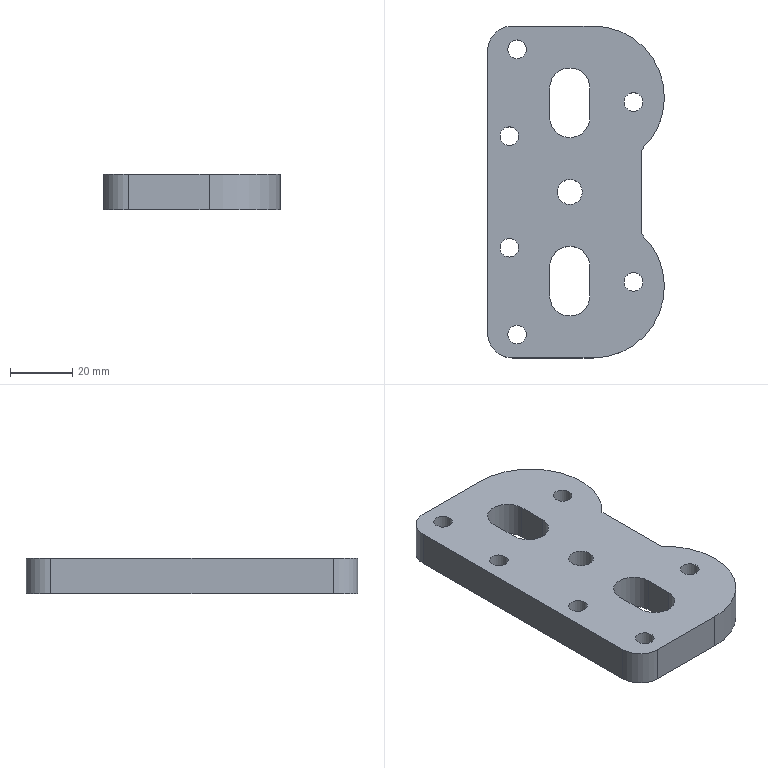Component | NX | UPPER_TOP_PLATE | 1 solid | 25 faces | volume 55554 mm3 | cylinder 15 | plane 10 | commonest cylinder face diameters 6 x6 13 x4 46 x2 16 x2 8 x1